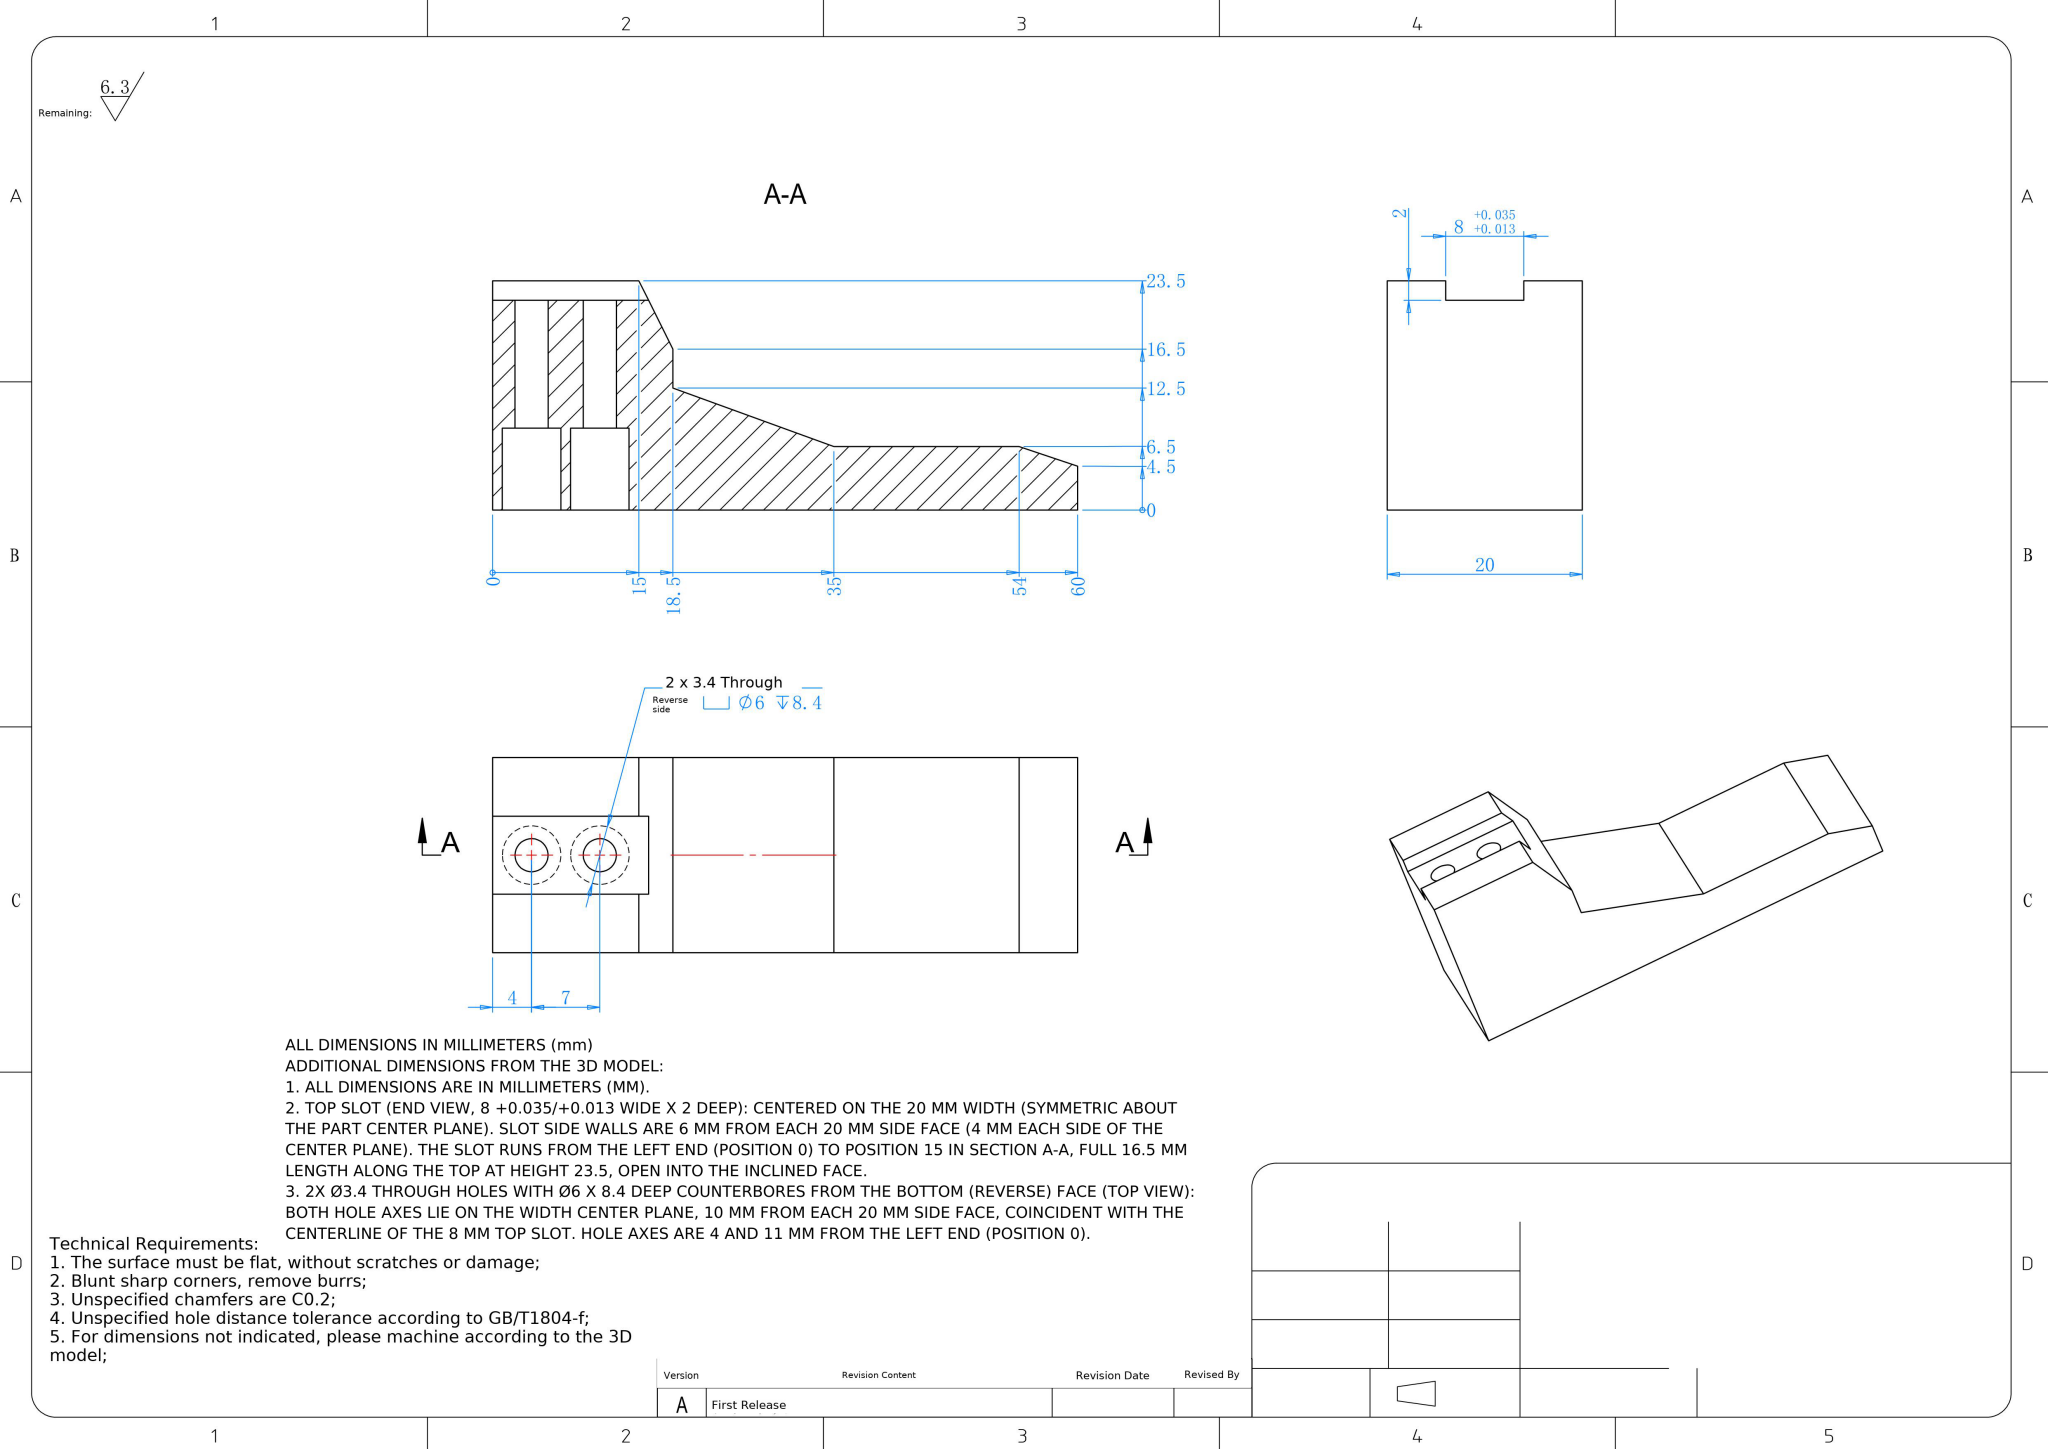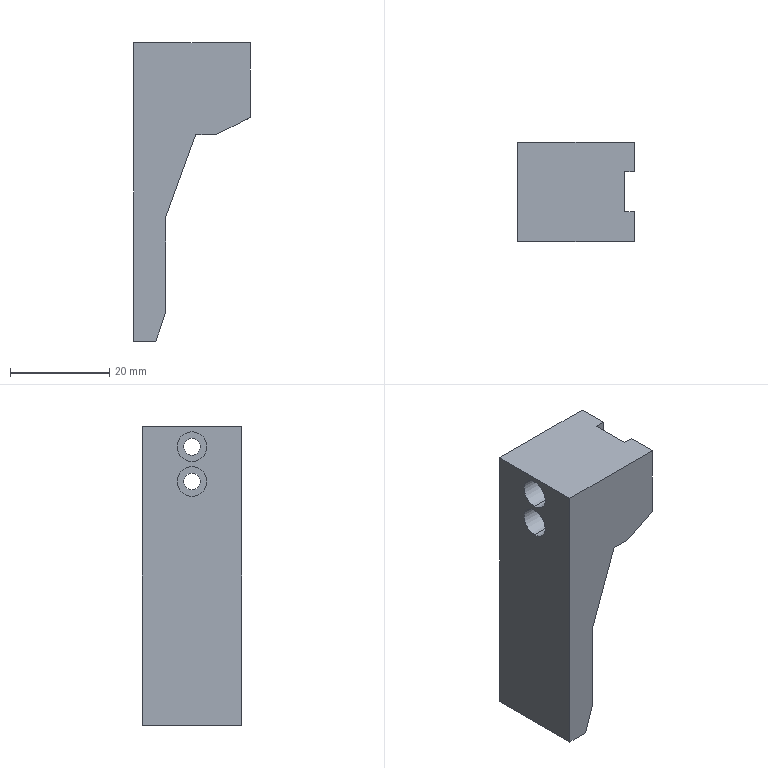Part | NX | mm | Stepped Dual-Bore Angled Mounting Bracket | 1 solid | 25 faces | box 23.5 x 20 x 60 mm | volume 13754 mm3 | plane 17 | cylinder 8 | commonest cylinder face diameters 6 x4 3.4 x4
STEP:
#1=COLOUR_RGB('',0.7922,0.8196,0.9333);
#2=FILL_AREA_STYLE_COLOUR('',#1);
#3=FILL_AREA_STYLE('',(#2));
#4=SURFACE_STYLE_FILL_AREA(#3);
#5=SURFACE_SIDE_STYLE('',(#4));
#6=SURFACE_STYLE_USAGE(.BOTH.,#5);
#7=PRESENTATION_STYLE_ASSIGNMENT((#6));
#8=CARTESIAN_POINT('',(8.4,0.,41.));
#9=VERTEX_POINT('',#8);
#10=CARTESIAN_POINT('',(8.4,0.,47.));
#11=VERTEX_POINT('',#10);
#12=CARTESIAN_POINT('',(8.4,0.,44.));
#13=DIRECTION('',(-1.,0.,0.));
#14=DIRECTION('',(0.,0.,1.));
#15=AXIS2_PLACEMENT_3D('',#12,#13,#14);
#16=CIRCLE('',#15,3.);
#17=EDGE_CURVE('',#9,#11,#16,.T.);
#18=ORIENTED_EDGE('',*,*,#17,.F.);
#19=CARTESIAN_POINT('',(0.,0.,41.));
#20=VERTEX_POINT('',#19);
#21=CARTESIAN_POINT('',(0.,0.,41.));
#22=DIRECTION('',(-1.,0.,0.));
#23=VECTOR('',#22,1000.);
#24=LINE('',#21,#23);
#25=EDGE_CURVE('',#9,#20,#24,.T.);
#26=ORIENTED_EDGE('',*,*,#25,.T.);
#27=CARTESIAN_POINT('',(0.,0.,47.));
#28=VERTEX_POINT('',#27);
#29=CARTESIAN_POINT('',(0.,0.,44.));
#30=DIRECTION('',(-1.,0.,0.));
#31=DIRECTION('',(0.,0.,1.));
#32=AXIS2_PLACEMENT_3D('',#29,#30,#31);
#33=CIRCLE('',#32,3.);
#34=EDGE_CURVE('',#20,#28,#33,.T.);
#35=ORIENTED_EDGE('',*,*,#34,.T.);
#36=CARTESIAN_POINT('',(0.,0.,47.));
#37=DIRECTION('',(-1.,0.,0.));
#38=VECTOR('',#37,1000.);
#39=LINE('',#36,#38);
#40=EDGE_CURVE('',#11,#28,#39,.T.);
#41=ORIENTED_EDGE('',*,*,#40,.F.);
#42=EDGE_LOOP('',(#18,#26,#35,#41));
#43=FACE_OUTER_BOUND('',#42,.T.);
#44=CARTESIAN_POINT('',(0.,0.,44.));
#45=DIRECTION('',(-1.,0.,0.));
#46=DIRECTION('',(0.,0.,1.));
#47=AXIS2_PLACEMENT_3D('',#44,#45,#46);
#48=CYLINDRICAL_SURFACE('',#47,3.);
#49=ADVANCED_FACE('',(#43),#48,.F.);
#50=CARTESIAN_POINT('',(21.5,0.,42.3));
#51=VERTEX_POINT('',#50);
#52=CARTESIAN_POINT('',(21.5,0.,45.7));
#53=VERTEX_POINT('',#52);
#54=CARTESIAN_POINT('',(21.5,0.,44.));
#55=DIRECTION('',(-1.,0.,0.));
#56=DIRECTION('',(0.,0.,1.));
#57=AXIS2_PLACEMENT_3D('',#54,#55,#56);
#58=CIRCLE('',#57,1.7);
#59=EDGE_CURVE('',#51,#53,#58,.T.);
#60=ORIENTED_EDGE('',*,*,#59,.F.);
#61=CARTESIAN_POINT('',(8.4,0.,42.3));
#62=VERTEX_POINT('',#61);
#63=CARTESIAN_POINT('',(0.,0.,42.3));
#64=DIRECTION('',(-1.,0.,0.));
#65=VECTOR('',#64,1000.);
#66=LINE('',#63,#65);
#67=EDGE_CURVE('',#51,#62,#66,.T.);
#68=ORIENTED_EDGE('',*,*,#67,.T.);
#69=CARTESIAN_POINT('',(8.4,0.,45.7));
#70=VERTEX_POINT('',#69);
#71=CARTESIAN_POINT('',(8.4,0.,44.));
#72=DIRECTION('',(-1.,0.,0.));
#73=DIRECTION('',(0.,0.,1.));
#74=AXIS2_PLACEMENT_3D('',#71,#72,#73);
#75=CIRCLE('',#74,1.7);
#76=EDGE_CURVE('',#62,#70,#75,.T.);
#77=ORIENTED_EDGE('',*,*,#76,.T.);
#78=CARTESIAN_POINT('',(0.,0.,45.7));
#79=DIRECTION('',(-1.,0.,0.));
#80=VECTOR('',#79,1000.);
#81=LINE('',#78,#80);
#82=EDGE_CURVE('',#53,#70,#81,.T.);
#83=ORIENTED_EDGE('',*,*,#82,.F.);
#84=EDGE_LOOP('',(#60,#68,#77,#83));
#85=FACE_OUTER_BOUND('',#84,.T.);
#86=CARTESIAN_POINT('',(0.,0.,44.));
#87=DIRECTION('',(-1.,0.,0.));
#88=DIRECTION('',(0.,0.,1.));
#89=AXIS2_PLACEMENT_3D('',#86,#87,#88);
#90=CYLINDRICAL_SURFACE('',#89,1.7);
#91=ADVANCED_FACE('',(#85),#90,.F.);
#92=CARTESIAN_POINT('',(8.4,0.,34.));
#93=VERTEX_POINT('',#92);
#94=CARTESIAN_POINT('',(8.4,0.,40.));
#95=VERTEX_POINT('',#94);
#96=CARTESIAN_POINT('',(8.4,0.,37.));
#97=DIRECTION('',(-1.,0.,0.));
#98=DIRECTION('',(0.,0.,1.));
#99=AXIS2_PLACEMENT_3D('',#96,#97,#98);
#100=CIRCLE('',#99,3.);
#101=EDGE_CURVE('',#93,#95,#100,.T.);
#102=ORIENTED_EDGE('',*,*,#101,.F.);
#103=CARTESIAN_POINT('',(0.,0.,34.));
#104=VERTEX_POINT('',#103);
#105=CARTESIAN_POINT('',(0.,0.,34.));
#106=DIRECTION('',(-1.,0.,0.));
#107=VECTOR('',#106,1000.);
#108=LINE('',#105,#107);
#109=EDGE_CURVE('',#93,#104,#108,.T.);
#110=ORIENTED_EDGE('',*,*,#109,.T.);
#111=CARTESIAN_POINT('',(0.,0.,40.));
#112=VERTEX_POINT('',#111);
#113=CARTESIAN_POINT('',(0.,0.,37.));
#114=DIRECTION('',(-1.,0.,0.));
#115=DIRECTION('',(0.,0.,1.));
#116=AXIS2_PLACEMENT_3D('',#113,#114,#115);
#117=CIRCLE('',#116,3.);
#118=EDGE_CURVE('',#104,#112,#117,.T.);
#119=ORIENTED_EDGE('',*,*,#118,.T.);
#120=CARTESIAN_POINT('',(0.,0.,40.));
#121=DIRECTION('',(-1.,0.,0.));
#122=VECTOR('',#121,1000.);
#123=LINE('',#120,#122);
#124=EDGE_CURVE('',#95,#112,#123,.T.);
#125=ORIENTED_EDGE('',*,*,#124,.F.);
#126=EDGE_LOOP('',(#102,#110,#119,#125));
#127=FACE_OUTER_BOUND('',#126,.T.);
#128=CARTESIAN_POINT('',(0.,0.,37.));
#129=DIRECTION('',(-1.,0.,0.));
#130=DIRECTION('',(0.,0.,1.));
#131=AXIS2_PLACEMENT_3D('',#128,#129,#130);
#132=CYLINDRICAL_SURFACE('',#131,3.);
#133=ADVANCED_FACE('',(#127),#132,.F.);
#134=CARTESIAN_POINT('',(21.5,0.,35.3));
#135=VERTEX_POINT('',#134);
#136=CARTESIAN_POINT('',(21.5,0.,38.7));
#137=VERTEX_POINT('',#136);
#138=CARTESIAN_POINT('',(21.5,0.,37.));
#139=DIRECTION('',(-1.,0.,0.));
#140=DIRECTION('',(0.,0.,1.));
#141=AXIS2_PLACEMENT_3D('',#138,#139,#140);
#142=CIRCLE('',#141,1.7);
#143=EDGE_CURVE('',#135,#137,#142,.T.);
#144=ORIENTED_EDGE('',*,*,#143,.F.);
#145=CARTESIAN_POINT('',(8.4,0.,35.3));
#146=VERTEX_POINT('',#145);
#147=CARTESIAN_POINT('',(0.,0.,35.3));
#148=DIRECTION('',(-1.,0.,0.));
#149=VECTOR('',#148,1000.);
#150=LINE('',#147,#149);
#151=EDGE_CURVE('',#135,#146,#150,.T.);
#152=ORIENTED_EDGE('',*,*,#151,.T.);
#153=CARTESIAN_POINT('',(8.4,0.,38.7));
#154=VERTEX_POINT('',#153);
#155=CARTESIAN_POINT('',(8.4,0.,37.));
#156=DIRECTION('',(-1.,0.,0.));
#157=DIRECTION('',(0.,0.,1.));
#158=AXIS2_PLACEMENT_3D('',#155,#156,#157);
#159=CIRCLE('',#158,1.7);
#160=EDGE_CURVE('',#146,#154,#159,.T.);
#161=ORIENTED_EDGE('',*,*,#160,.T.);
#162=CARTESIAN_POINT('',(0.,0.,38.7));
#163=DIRECTION('',(-1.,0.,0.));
#164=VECTOR('',#163,1000.);
#165=LINE('',#162,#164);
#166=EDGE_CURVE('',#137,#154,#165,.T.);
#167=ORIENTED_EDGE('',*,*,#166,.F.);
#168=EDGE_LOOP('',(#144,#152,#161,#167));
#169=FACE_OUTER_BOUND('',#168,.T.);
#170=CARTESIAN_POINT('',(0.,0.,37.));
#171=DIRECTION('',(-1.,0.,0.));
#172=DIRECTION('',(0.,0.,1.));
#173=AXIS2_PLACEMENT_3D('',#170,#171,#172);
#174=CYLINDRICAL_SURFACE('',#173,1.7);
#175=ADVANCED_FACE('',(#169),#174,.F.);
#176=CARTESIAN_POINT('',(23.5,-4.,33.));
#177=VERTEX_POINT('',#176);
#178=CARTESIAN_POINT('',(23.5,-10.,33.));
#179=VERTEX_POINT('',#178);
#180=CARTESIAN_POINT('',(23.5,10.,33.));
#181=DIRECTION('',(0.,-1.,0.));
#182=VECTOR('',#181,1000.);
#183=LINE('',#180,#182);
#184=EDGE_CURVE('',#177,#179,#183,.T.);
#185=ORIENTED_EDGE('',*,*,#184,.F.);
#186=CARTESIAN_POINT('',(23.5,-4.,48.));
#187=VERTEX_POINT('',#186);
#188=CARTESIAN_POINT('',(23.5,-4.,33.));
#189=DIRECTION('',(0.,0.,1.));
#190=VECTOR('',#189,1000.);
#191=LINE('',#188,#190);
#192=EDGE_CURVE('',#177,#187,#191,.T.);
#193=ORIENTED_EDGE('',*,*,#192,.T.);
#194=CARTESIAN_POINT('',(23.5,-10.,48.));
#195=VERTEX_POINT('',#194);
#196=CARTESIAN_POINT('',(23.5,10.,48.));
#197=DIRECTION('',(0.,-1.,0.));
#198=VECTOR('',#197,1000.);
#199=LINE('',#196,#198);
#200=EDGE_CURVE('',#187,#195,#199,.T.);
#201=ORIENTED_EDGE('',*,*,#200,.T.);
#202=CARTESIAN_POINT('',(23.5,-10.,33.));
#203=DIRECTION('',(-0.,0.,-1.));
#204=VECTOR('',#203,1000.);
#205=LINE('',#202,#204);
#206=EDGE_CURVE('',#195,#179,#205,.T.);
#207=ORIENTED_EDGE('',*,*,#206,.T.);
#208=EDGE_LOOP('',(#185,#193,#201,#207));
#209=FACE_OUTER_BOUND('',#208,.T.);
#210=CARTESIAN_POINT('',(23.5,10.,33.));
#211=DIRECTION('',(-1.,0.,0.));
#212=DIRECTION('',(0.,0.,1.));
#213=AXIS2_PLACEMENT_3D('',#210,#211,#212);
#214=PLANE('',#213);
#215=ADVANCED_FACE('',(#209),#214,.F.);
#216=CARTESIAN_POINT('',(0.,0.,44.));
#217=DIRECTION('',(-1.,0.,0.));
#218=DIRECTION('',(0.,0.,1.));
#219=AXIS2_PLACEMENT_3D('',#216,#217,#218);
#220=CIRCLE('',#219,3.);
#221=EDGE_CURVE('',#28,#20,#220,.T.);
#222=ORIENTED_EDGE('',*,*,#221,.F.);
#223=ORIENTED_EDGE('',*,*,#34,.F.);
#224=EDGE_LOOP('',(#222,#223));
#225=FACE_BOUND('',#224,.T.);
#226=CARTESIAN_POINT('',(0.,0.,37.));
#227=DIRECTION('',(-1.,0.,0.));
#228=DIRECTION('',(0.,0.,1.));
#229=AXIS2_PLACEMENT_3D('',#226,#227,#228);
#230=CIRCLE('',#229,3.);
#231=EDGE_CURVE('',#112,#104,#230,.T.);
#232=ORIENTED_EDGE('',*,*,#231,.F.);
#233=ORIENTED_EDGE('',*,*,#118,.F.);
#234=EDGE_LOOP('',(#232,#233));
#235=FACE_BOUND('',#234,.T.);
#236=CARTESIAN_POINT('',(0.,-10.,-12.));
#237=VERTEX_POINT('',#236);
#238=CARTESIAN_POINT('',(0.,-10.,48.));
#239=VERTEX_POINT('',#238);
#240=CARTESIAN_POINT('',(0.,-10.,48.));
#241=DIRECTION('',(0.,0.,1.));
#242=VECTOR('',#241,1000.);
#243=LINE('',#240,#242);
#244=EDGE_CURVE('',#237,#239,#243,.T.);
#245=ORIENTED_EDGE('',*,*,#244,.T.);
#246=CARTESIAN_POINT('',(0.,10.,48.));
#247=VERTEX_POINT('',#246);
#248=CARTESIAN_POINT('',(0.,10.,48.));
#249=DIRECTION('',(0.,-1.,0.));
#250=VECTOR('',#249,1000.);
#251=LINE('',#248,#250);
#252=EDGE_CURVE('',#247,#239,#251,.T.);
#253=ORIENTED_EDGE('',*,*,#252,.F.);
#254=CARTESIAN_POINT('',(0.,10.,-12.));
#255=VERTEX_POINT('',#254);
#256=CARTESIAN_POINT('',(0.,10.,48.));
#257=DIRECTION('',(0.,0.,1.));
#258=VECTOR('',#257,1000.);
#259=LINE('',#256,#258);
#260=EDGE_CURVE('',#255,#247,#259,.T.);
#261=ORIENTED_EDGE('',*,*,#260,.F.);
#262=CARTESIAN_POINT('',(0.,10.,-12.));
#263=DIRECTION('',(0.,-1.,0.));
#264=VECTOR('',#263,1000.);
#265=LINE('',#262,#264);
#266=EDGE_CURVE('',#255,#237,#265,.T.);
#267=ORIENTED_EDGE('',*,*,#266,.T.);
#268=EDGE_LOOP('',(#245,#253,#261,#267));
#269=FACE_OUTER_BOUND('',#268,.T.);
#270=CARTESIAN_POINT('',(0.,10.,48.));
#271=DIRECTION('',(1.,0.,0.));
#272=DIRECTION('',(0.,0.,-1.));
#273=AXIS2_PLACEMENT_3D('',#270,#271,#272);
#274=PLANE('',#273);
#275=ADVANCED_FACE('',(#225,#235,#269),#274,.F.);
#276=ORIENTED_EDGE('',*,*,#200,.F.);
#277=CARTESIAN_POINT('',(21.5,-4.,48.));
#278=VERTEX_POINT('',#277);
#279=CARTESIAN_POINT('',(21.5,-4.,48.));
#280=DIRECTION('',(1.,0.,0.));
#281=VECTOR('',#280,1000.);
#282=LINE('',#279,#281);
#283=EDGE_CURVE('',#278,#187,#282,.T.);
#284=ORIENTED_EDGE('',*,*,#283,.F.);
#285=CARTESIAN_POINT('',(21.5,4.,48.));
#286=VERTEX_POINT('',#285);
#287=CARTESIAN_POINT('',(21.5,-4.,48.));
#288=DIRECTION('',(0.,-1.,0.));
#289=VECTOR('',#288,1000.);
#290=LINE('',#287,#289);
#291=EDGE_CURVE('',#286,#278,#290,.T.);
#292=ORIENTED_EDGE('',*,*,#291,.F.);
#293=CARTESIAN_POINT('',(23.5,4.,48.));
#294=VERTEX_POINT('',#293);
#295=CARTESIAN_POINT('',(21.5,4.,48.));
#296=DIRECTION('',(-1.,0.,0.));
#297=VECTOR('',#296,1000.);
#298=LINE('',#295,#297);
#299=EDGE_CURVE('',#294,#286,#298,.T.);
#300=ORIENTED_EDGE('',*,*,#299,.F.);
#301=CARTESIAN_POINT('',(23.5,10.,48.));
#302=VERTEX_POINT('',#301);
#303=CARTESIAN_POINT('',(23.5,10.,48.));
#304=DIRECTION('',(0.,-1.,0.));
#305=VECTOR('',#304,1000.);
#306=LINE('',#303,#305);
#307=EDGE_CURVE('',#302,#294,#306,.T.);
#308=ORIENTED_EDGE('',*,*,#307,.F.);
#309=CARTESIAN_POINT('',(23.5,10.,48.));
#310=DIRECTION('',(1.,0.,0.));
#311=VECTOR('',#310,1000.);
#312=LINE('',#309,#311);
#313=EDGE_CURVE('',#247,#302,#312,.T.);
#314=ORIENTED_EDGE('',*,*,#313,.F.);
#315=ORIENTED_EDGE('',*,*,#252,.T.);
#316=CARTESIAN_POINT('',(23.5,-10.,48.));
#317=DIRECTION('',(1.,0.,0.));
#318=VECTOR('',#317,1000.);
#319=LINE('',#316,#318);
#320=EDGE_CURVE('',#239,#195,#319,.T.);
#321=ORIENTED_EDGE('',*,*,#320,.T.);
#322=EDGE_LOOP('',(#276,#284,#292,#300,#308,#314,#315,#321));
#323=FACE_OUTER_BOUND('',#322,.T.);
#324=CARTESIAN_POINT('',(23.5,10.,48.));
#325=DIRECTION('',(0.,0.,-1.));
#326=DIRECTION('',(-1.,0.,0.));
#327=AXIS2_PLACEMENT_3D('',#324,#325,#326);
#328=PLANE('',#327);
#329=ADVANCED_FACE('',(#323),#328,.F.);
#330=ORIENTED_EDGE('',*,*,#307,.T.);
#331=CARTESIAN_POINT('',(23.5,4.,33.));
#332=VERTEX_POINT('',#331);
#333=CARTESIAN_POINT('',(23.5,4.,33.));
#334=DIRECTION('',(-0.,0.,-1.));
#335=VECTOR('',#334,1000.);
#336=LINE('',#333,#335);
#337=EDGE_CURVE('',#294,#332,#336,.T.);
#338=ORIENTED_EDGE('',*,*,#337,.T.);
#339=CARTESIAN_POINT('',(23.5,10.,33.));
#340=VERTEX_POINT('',#339);
#341=CARTESIAN_POINT('',(23.5,10.,33.));
#342=DIRECTION('',(0.,-1.,0.));
#343=VECTOR('',#342,1000.);
#344=LINE('',#341,#343);
#345=EDGE_CURVE('',#340,#332,#344,.T.);
#346=ORIENTED_EDGE('',*,*,#345,.F.);
#347=CARTESIAN_POINT('',(23.5,10.,33.));
#348=DIRECTION('',(-0.,0.,-1.));
#349=VECTOR('',#348,1000.);
#350=LINE('',#347,#349);
#351=EDGE_CURVE('',#302,#340,#350,.T.);
#352=ORIENTED_EDGE('',*,*,#351,.F.);
#353=EDGE_LOOP('',(#330,#338,#346,#352));
#354=FACE_OUTER_BOUND('',#353,.T.);
#355=CARTESIAN_POINT('',(23.5,10.,33.));
#356=DIRECTION('',(-1.,0.,0.));
#357=DIRECTION('',(0.,0.,1.));
#358=AXIS2_PLACEMENT_3D('',#355,#356,#357);
#359=PLANE('',#358);
#360=ADVANCED_FACE('',(#354),#359,.F.);
#361=CARTESIAN_POINT('',(21.5,4.,32.));
#362=VERTEX_POINT('',#361);
#363=CARTESIAN_POINT('',(21.5,-4.,32.));
#364=VERTEX_POINT('',#363);
#365=CARTESIAN_POINT('',(21.5,10.,32.));
#366=DIRECTION('',(0.,-1.,0.));
#367=VECTOR('',#366,1000.);
#368=LINE('',#365,#367);
#369=EDGE_CURVE('',#362,#364,#368,.T.);
#370=ORIENTED_EDGE('',*,*,#369,.T.);
#371=CARTESIAN_POINT('',(23.5,-4.,33.));
#372=DIRECTION('',(0.8944,0.,0.4472));
#373=VECTOR('',#372,1000.);
#374=LINE('',#371,#373);
#375=EDGE_CURVE('',#364,#177,#374,.T.);
#376=ORIENTED_EDGE('',*,*,#375,.T.);
#377=ORIENTED_EDGE('',*,*,#184,.T.);
#378=CARTESIAN_POINT('',(16.5,-10.,29.5));
#379=VERTEX_POINT('',#378);
#380=CARTESIAN_POINT('',(23.5,-10.,33.));
#381=DIRECTION('',(-0.8944,0.,-0.4472));
#382=VECTOR('',#381,1000.);
#383=LINE('',#380,#382);
#384=EDGE_CURVE('',#179,#379,#383,.T.);
#385=ORIENTED_EDGE('',*,*,#384,.T.);
#386=CARTESIAN_POINT('',(16.5,10.,29.5));
#387=VERTEX_POINT('',#386);
#388=CARTESIAN_POINT('',(16.5,10.,29.5));
#389=DIRECTION('',(0.,-1.,0.));
#390=VECTOR('',#389,1000.);
#391=LINE('',#388,#390);
#392=EDGE_CURVE('',#387,#379,#391,.T.);
#393=ORIENTED_EDGE('',*,*,#392,.F.);
#394=CARTESIAN_POINT('',(23.5,10.,33.));
#395=DIRECTION('',(-0.8944,0.,-0.4472));
#396=VECTOR('',#395,1000.);
#397=LINE('',#394,#396);
#398=EDGE_CURVE('',#340,#387,#397,.T.);
#399=ORIENTED_EDGE('',*,*,#398,.F.);
#400=ORIENTED_EDGE('',*,*,#345,.T.);
#401=CARTESIAN_POINT('',(23.5,4.,33.));
#402=DIRECTION('',(-0.8944,0.,-0.4472));
#403=VECTOR('',#402,1000.);
#404=LINE('',#401,#403);
#405=EDGE_CURVE('',#332,#362,#404,.T.);
#406=ORIENTED_EDGE('',*,*,#405,.T.);
#407=EDGE_LOOP('',(#370,#376,#377,#385,#393,#399,#400,#406));
#408=FACE_OUTER_BOUND('',#407,.T.);
#409=CARTESIAN_POINT('',(23.5,10.,33.));
#410=DIRECTION('',(-0.4472,0.,0.8944));
#411=DIRECTION('',(0.8944,0.,0.4472));
#412=AXIS2_PLACEMENT_3D('',#409,#410,#411);
#413=PLANE('',#412);
#414=ADVANCED_FACE('',(#408),#413,.F.);
#415=CARTESIAN_POINT('',(12.5,-10.,29.5));
#416=VERTEX_POINT('',#415);
#417=CARTESIAN_POINT('',(16.5,-10.,29.5));
#418=DIRECTION('',(-1.,0.,0.));
#419=VECTOR('',#418,1000.);
#420=LINE('',#417,#419);
#421=EDGE_CURVE('',#379,#416,#420,.T.);
#422=ORIENTED_EDGE('',*,*,#421,.T.);
#423=CARTESIAN_POINT('',(12.5,10.,29.5));
#424=VERTEX_POINT('',#423);
#425=CARTESIAN_POINT('',(12.5,10.,29.5));
#426=DIRECTION('',(0.,-1.,0.));
#427=VECTOR('',#426,1000.);
#428=LINE('',#425,#427);
#429=EDGE_CURVE('',#424,#416,#428,.T.);
#430=ORIENTED_EDGE('',*,*,#429,.F.);
#431=CARTESIAN_POINT('',(16.5,10.,29.5));
#432=DIRECTION('',(-1.,0.,0.));
#433=VECTOR('',#432,1000.);
#434=LINE('',#431,#433);
#435=EDGE_CURVE('',#387,#424,#434,.T.);
#436=ORIENTED_EDGE('',*,*,#435,.F.);
#437=ORIENTED_EDGE('',*,*,#392,.T.);
#438=EDGE_LOOP('',(#422,#430,#436,#437));
#439=FACE_OUTER_BOUND('',#438,.T.);
#440=CARTESIAN_POINT('',(16.5,10.,29.5));
#441=DIRECTION('',(0.,0.,1.));
#442=DIRECTION('',(1.,0.,0.));
#443=AXIS2_PLACEMENT_3D('',#440,#441,#442);
#444=PLANE('',#443);
#445=ADVANCED_FACE('',(#439),#444,.F.);
#446=CARTESIAN_POINT('',(6.5,-10.,13.));
#447=VERTEX_POINT('',#446);
#448=CARTESIAN_POINT('',(12.5,-10.,29.5));
#449=DIRECTION('',(-0.3417,0.,-0.9398));
#450=VECTOR('',#449,1000.);
#451=LINE('',#448,#450);
#452=EDGE_CURVE('',#416,#447,#451,.T.);
#453=ORIENTED_EDGE('',*,*,#452,.T.);
#454=CARTESIAN_POINT('',(6.5,10.,13.));
#455=VERTEX_POINT('',#454);
#456=CARTESIAN_POINT('',(6.5,10.,13.));
#457=DIRECTION('',(0.,-1.,0.));
#458=VECTOR('',#457,1000.);
#459=LINE('',#456,#458);
#460=EDGE_CURVE('',#455,#447,#459,.T.);
#461=ORIENTED_EDGE('',*,*,#460,.F.);
#462=CARTESIAN_POINT('',(12.5,10.,29.5));
#463=DIRECTION('',(-0.3417,0.,-0.9398));
#464=VECTOR('',#463,1000.);
#465=LINE('',#462,#464);
#466=EDGE_CURVE('',#424,#455,#465,.T.);
#467=ORIENTED_EDGE('',*,*,#466,.F.);
#468=ORIENTED_EDGE('',*,*,#429,.T.);
#469=EDGE_LOOP('',(#453,#461,#467,#468));
#470=FACE_OUTER_BOUND('',#469,.T.);
#471=CARTESIAN_POINT('',(12.5,10.,29.5));
#472=DIRECTION('',(-0.9398,0.,0.3417));
#473=DIRECTION('',(0.3417,0.,0.9398));
#474=AXIS2_PLACEMENT_3D('',#471,#472,#473);
#475=PLANE('',#474);
#476=ADVANCED_FACE('',(#470),#475,.F.);
#477=CARTESIAN_POINT('',(6.5,-10.,-6.));
#478=VERTEX_POINT('',#477);
#479=CARTESIAN_POINT('',(6.5,-10.,-12.));
#480=DIRECTION('',(0.,0.,-1.));
#481=VECTOR('',#480,1000.);
#482=LINE('',#479,#481);
#483=EDGE_CURVE('',#447,#478,#482,.T.);
#484=ORIENTED_EDGE('',*,*,#483,.T.);
#485=CARTESIAN_POINT('',(6.5,10.,-6.));
#486=VERTEX_POINT('',#485);
#487=CARTESIAN_POINT('',(6.5,10.,-6.));
#488=DIRECTION('',(0.,-1.,0.));
#489=VECTOR('',#488,1000.);
#490=LINE('',#487,#489);
#491=EDGE_CURVE('',#486,#478,#490,.T.);
#492=ORIENTED_EDGE('',*,*,#491,.F.);
#493=CARTESIAN_POINT('',(6.5,10.,-12.));
#494=DIRECTION('',(0.,0.,-1.));
#495=VECTOR('',#494,1000.);
#496=LINE('',#493,#495);
#497=EDGE_CURVE('',#455,#486,#496,.T.);
#498=ORIENTED_EDGE('',*,*,#497,.F.);
#499=ORIENTED_EDGE('',*,*,#460,.T.);
#500=EDGE_LOOP('',(#484,#492,#498,#499));
#501=FACE_OUTER_BOUND('',#500,.T.);
#502=CARTESIAN_POINT('',(6.5,10.,-12.));
#503=DIRECTION('',(-1.,0.,-0.));
#504=DIRECTION('',(-0.,0.,1.));
#505=AXIS2_PLACEMENT_3D('',#502,#503,#504);
#506=PLANE('',#505);
#507=ADVANCED_FACE('',(#501),#506,.F.);
#508=CARTESIAN_POINT('',(4.5,10.,-12.));
#509=VERTEX_POINT('',#508);
#510=CARTESIAN_POINT('',(0.,10.,-12.));
#511=DIRECTION('',(-1.,0.,0.));
#512=VECTOR('',#511,1000.);
#513=LINE('',#510,#512);
#514=EDGE_CURVE('',#509,#255,#513,.T.);
#515=ORIENTED_EDGE('',*,*,#514,.F.);
#516=CARTESIAN_POINT('',(4.5,-10.,-12.));
#517=VERTEX_POINT('',#516);
#518=CARTESIAN_POINT('',(4.5,10.,-12.));
#519=DIRECTION('',(0.,-1.,0.));
#520=VECTOR('',#519,1000.);
#521=LINE('',#518,#520);
#522=EDGE_CURVE('',#509,#517,#521,.T.);
#523=ORIENTED_EDGE('',*,*,#522,.T.);
#524=CARTESIAN_POINT('',(0.,-10.,-12.));
#525=DIRECTION('',(-1.,0.,0.));
#526=VECTOR('',#525,1000.);
#527=LINE('',#524,#526);
#528=EDGE_CURVE('',#517,#237,#527,.T.);
#529=ORIENTED_EDGE('',*,*,#528,.T.);
#530=ORIENTED_EDGE('',*,*,#266,.F.);
#531=EDGE_LOOP('',(#515,#523,#529,#530));
#532=FACE_OUTER_BOUND('',#531,.T.);
#533=CARTESIAN_POINT('',(0.,10.,-12.));
#534=DIRECTION('',(0.,0.,1.));
#535=DIRECTION('',(1.,0.,-0.));
#536=AXIS2_PLACEMENT_3D('',#533,#534,#535);
#537=PLANE('',#536);
#538=ADVANCED_FACE('',(#532),#537,.F.);
#539=ORIENTED_EDGE('',*,*,#497,.T.);
#540=CARTESIAN_POINT('',(4.5,10.,-12.));
#541=DIRECTION('',(-0.3162,0.,-0.9487));
#542=VECTOR('',#541,1000.);
#543=LINE('',#540,#542);
#544=EDGE_CURVE('',#486,#509,#543,.T.);
#545=ORIENTED_EDGE('',*,*,#544,.T.);
#546=ORIENTED_EDGE('',*,*,#514,.T.);
#547=ORIENTED_EDGE('',*,*,#260,.T.);
#548=ORIENTED_EDGE('',*,*,#313,.T.);
#549=ORIENTED_EDGE('',*,*,#351,.T.);
#550=ORIENTED_EDGE('',*,*,#398,.T.);
#551=ORIENTED_EDGE('',*,*,#435,.T.);
#552=ORIENTED_EDGE('',*,*,#466,.T.);
#553=EDGE_LOOP('',(#539,#545,#546,#547,#548,#549,#550,#551,#552));
#554=FACE_OUTER_BOUND('',#553,.T.);
#555=CARTESIAN_POINT('',(0.,10.,0.));
#556=DIRECTION('',(0.,-1.,0.));
#557=DIRECTION('',(0.,0.,-1.));
#558=AXIS2_PLACEMENT_3D('',#555,#556,#557);
#559=PLANE('',#558);
#560=ADVANCED_FACE('',(#554),#559,.F.);
#561=CARTESIAN_POINT('',(4.5,-10.,-12.));
#562=DIRECTION('',(-0.3162,0.,-0.9487));
#563=VECTOR('',#562,1000.);
#564=LINE('',#561,#563);
#565=EDGE_CURVE('',#478,#517,#564,.T.);
#566=ORIENTED_EDGE('',*,*,#565,.F.);
#567=ORIENTED_EDGE('',*,*,#483,.F.);
#568=ORIENTED_EDGE('',*,*,#452,.F.);
#569=ORIENTED_EDGE('',*,*,#421,.F.);
#570=ORIENTED_EDGE('',*,*,#384,.F.);
#571=ORIENTED_EDGE('',*,*,#206,.F.);
#572=ORIENTED_EDGE('',*,*,#320,.F.);
#573=ORIENTED_EDGE('',*,*,#244,.F.);
#574=ORIENTED_EDGE('',*,*,#528,.F.);
#575=EDGE_LOOP('',(#566,#567,#568,#569,#570,#571,#572,#573,#574));
#576=FACE_OUTER_BOUND('',#575,.T.);
#577=CARTESIAN_POINT('',(0.,-10.,0.));
#578=DIRECTION('',(0.,-1.,0.));
#579=DIRECTION('',(0.,0.,-1.));
#580=AXIS2_PLACEMENT_3D('',#577,#578,#579);
#581=PLANE('',#580);
#582=ADVANCED_FACE('',(#576),#581,.T.);
#583=ORIENTED_EDGE('',*,*,#375,.F.);
#584=CARTESIAN_POINT('',(21.5,-4.,-12.));
#585=DIRECTION('',(0.,0.,1.));
#586=VECTOR('',#585,1000.);
#587=LINE('',#584,#586);
#588=EDGE_CURVE('',#364,#278,#587,.T.);
#589=ORIENTED_EDGE('',*,*,#588,.T.);
#590=ORIENTED_EDGE('',*,*,#283,.T.);
#591=ORIENTED_EDGE('',*,*,#192,.F.);
#592=EDGE_LOOP('',(#583,#589,#590,#591));
#593=FACE_OUTER_BOUND('',#592,.T.);
#594=CARTESIAN_POINT('',(21.5,-4.,-12.));
#595=DIRECTION('',(0.,-1.,0.));
#596=DIRECTION('',(0.,0.,-1.));
#597=AXIS2_PLACEMENT_3D('',#594,#595,#596);
#598=PLANE('',#597);
#599=ADVANCED_FACE('',(#593),#598,.F.);
#600=CARTESIAN_POINT('',(21.5,0.,44.));
#601=DIRECTION('',(-1.,0.,0.));
#602=DIRECTION('',(0.,0.,1.));
#603=AXIS2_PLACEMENT_3D('',#600,#601,#602);
#604=CIRCLE('',#603,1.7);
#605=EDGE_CURVE('',#53,#51,#604,.T.);
#606=ORIENTED_EDGE('',*,*,#605,.T.);
#607=ORIENTED_EDGE('',*,*,#59,.T.);
#608=EDGE_LOOP('',(#606,#607));
#609=FACE_BOUND('',#608,.T.);
#610=CARTESIAN_POINT('',(21.5,0.,37.));
#611=DIRECTION('',(-1.,0.,0.));
#612=DIRECTION('',(0.,0.,1.));
#613=AXIS2_PLACEMENT_3D('',#610,#611,#612);
#614=CIRCLE('',#613,1.7);
#615=EDGE_CURVE('',#137,#135,#614,.T.);
#616=ORIENTED_EDGE('',*,*,#615,.T.);
#617=ORIENTED_EDGE('',*,*,#143,.T.);
#618=EDGE_LOOP('',(#616,#617));
#619=FACE_BOUND('',#618,.T.);
#620=CARTESIAN_POINT('',(21.5,4.,-12.));
#621=DIRECTION('',(0.,0.,1.));
#622=VECTOR('',#621,1000.);
#623=LINE('',#620,#622);
#624=EDGE_CURVE('',#362,#286,#623,.T.);
#625=ORIENTED_EDGE('',*,*,#624,.T.);
#626=ORIENTED_EDGE('',*,*,#291,.T.);
#627=ORIENTED_EDGE('',*,*,#588,.F.);
#628=ORIENTED_EDGE('',*,*,#369,.F.);
#629=EDGE_LOOP('',(#625,#626,#627,#628));
#630=FACE_OUTER_BOUND('',#629,.T.);
#631=CARTESIAN_POINT('',(21.5,-4.,-12.));
#632=DIRECTION('',(-1.,0.,0.));
#633=DIRECTION('',(0.,0.,1.));
#634=AXIS2_PLACEMENT_3D('',#631,#632,#633);
#635=PLANE('',#634);
#636=ADVANCED_FACE('',(#609,#619,#630),#635,.F.);
#637=ORIENTED_EDGE('',*,*,#299,.T.);
#638=ORIENTED_EDGE('',*,*,#624,.F.);
#639=ORIENTED_EDGE('',*,*,#405,.F.);
#640=ORIENTED_EDGE('',*,*,#337,.F.);
#641=EDGE_LOOP('',(#637,#638,#639,#640));
#642=FACE_OUTER_BOUND('',#641,.T.);
#643=CARTESIAN_POINT('',(21.5,4.,-12.));
#644=DIRECTION('',(0.,1.,0.));
#645=DIRECTION('',(0.,0.,1.));
#646=AXIS2_PLACEMENT_3D('',#643,#644,#645);
#647=PLANE('',#646);
#648=ADVANCED_FACE('',(#642),#647,.F.);
#649=ORIENTED_EDGE('',*,*,#151,.F.);
#650=ORIENTED_EDGE('',*,*,#615,.F.);
#651=ORIENTED_EDGE('',*,*,#166,.T.);
#652=CARTESIAN_POINT('',(8.4,0.,37.));
#653=DIRECTION('',(-1.,0.,0.));
#654=DIRECTION('',(0.,0.,1.));
#655=AXIS2_PLACEMENT_3D('',#652,#653,#654);
#656=CIRCLE('',#655,1.7);
#657=EDGE_CURVE('',#154,#146,#656,.T.);
#658=ORIENTED_EDGE('',*,*,#657,.T.);
#659=EDGE_LOOP('',(#649,#650,#651,#658));
#660=FACE_OUTER_BOUND('',#659,.T.);
#661=CARTESIAN_POINT('',(0.,0.,37.));
#662=DIRECTION('',(-1.,0.,0.));
#663=DIRECTION('',(0.,0.,1.));
#664=AXIS2_PLACEMENT_3D('',#661,#662,#663);
#665=CYLINDRICAL_SURFACE('',#664,1.7);
#666=ADVANCED_FACE('',(#660),#665,.F.);
#667=ORIENTED_EDGE('',*,*,#657,.F.);
#668=ORIENTED_EDGE('',*,*,#160,.F.);
#669=EDGE_LOOP('',(#667,#668));
#670=FACE_BOUND('',#669,.T.);
#671=CARTESIAN_POINT('',(8.4,0.,37.));
#672=DIRECTION('',(-1.,0.,0.));
#673=DIRECTION('',(0.,0.,1.));
#674=AXIS2_PLACEMENT_3D('',#671,#672,#673);
#675=CIRCLE('',#674,3.);
#676=EDGE_CURVE('',#95,#93,#675,.T.);
#677=ORIENTED_EDGE('',*,*,#676,.T.);
#678=ORIENTED_EDGE('',*,*,#101,.T.);
#679=EDGE_LOOP('',(#677,#678));
#680=FACE_OUTER_BOUND('',#679,.T.);
#681=CARTESIAN_POINT('',(8.4,1.7,37.));
#682=DIRECTION('',(1.,0.,0.));
#683=DIRECTION('',(0.,0.,-1.));
#684=AXIS2_PLACEMENT_3D('',#681,#682,#683);
#685=PLANE('',#684);
#686=ADVANCED_FACE('',(#670,#680),#685,.F.);
#687=ORIENTED_EDGE('',*,*,#109,.F.);
#688=ORIENTED_EDGE('',*,*,#676,.F.);
#689=ORIENTED_EDGE('',*,*,#124,.T.);
#690=ORIENTED_EDGE('',*,*,#231,.T.);
#691=EDGE_LOOP('',(#687,#688,#689,#690));
#692=FACE_OUTER_BOUND('',#691,.T.);
#693=CARTESIAN_POINT('',(0.,0.,37.));
#694=DIRECTION('',(-1.,0.,0.));
#695=DIRECTION('',(0.,0.,1.));
#696=AXIS2_PLACEMENT_3D('',#693,#694,#695);
#697=CYLINDRICAL_SURFACE('',#696,3.);
#698=ADVANCED_FACE('',(#692),#697,.F.);
#699=ORIENTED_EDGE('',*,*,#67,.F.);
#700=ORIENTED_EDGE('',*,*,#605,.F.);
#701=ORIENTED_EDGE('',*,*,#82,.T.);
#702=CARTESIAN_POINT('',(8.4,0.,44.));
#703=DIRECTION('',(-1.,0.,0.));
#704=DIRECTION('',(0.,0.,1.));
#705=AXIS2_PLACEMENT_3D('',#702,#703,#704);
#706=CIRCLE('',#705,1.7);
#707=EDGE_CURVE('',#70,#62,#706,.T.);
#708=ORIENTED_EDGE('',*,*,#707,.T.);
#709=EDGE_LOOP('',(#699,#700,#701,#708));
#710=FACE_OUTER_BOUND('',#709,.T.);
#711=CARTESIAN_POINT('',(0.,0.,44.));
#712=DIRECTION('',(-1.,0.,0.));
#713=DIRECTION('',(0.,0.,1.));
#714=AXIS2_PLACEMENT_3D('',#711,#712,#713);
#715=CYLINDRICAL_SURFACE('',#714,1.7);
#716=ADVANCED_FACE('',(#710),#715,.F.);
#717=ORIENTED_EDGE('',*,*,#707,.F.);
#718=ORIENTED_EDGE('',*,*,#76,.F.);
#719=EDGE_LOOP('',(#717,#718));
#720=FACE_BOUND('',#719,.T.);
#721=CARTESIAN_POINT('',(8.4,0.,44.));
#722=DIRECTION('',(-1.,0.,0.));
#723=DIRECTION('',(0.,0.,1.));
#724=AXIS2_PLACEMENT_3D('',#721,#722,#723);
#725=CIRCLE('',#724,3.);
#726=EDGE_CURVE('',#11,#9,#725,.T.);
#727=ORIENTED_EDGE('',*,*,#726,.T.);
#728=ORIENTED_EDGE('',*,*,#17,.T.);
#729=EDGE_LOOP('',(#727,#728));
#730=FACE_OUTER_BOUND('',#729,.T.);
#731=CARTESIAN_POINT('',(8.4,1.7,44.));
#732=DIRECTION('',(1.,0.,0.));
#733=DIRECTION('',(0.,0.,-1.));
#734=AXIS2_PLACEMENT_3D('',#731,#732,#733);
#735=PLANE('',#734);
#736=ADVANCED_FACE('',(#720,#730),#735,.F.);
#737=ORIENTED_EDGE('',*,*,#25,.F.);
#738=ORIENTED_EDGE('',*,*,#726,.F.);
#739=ORIENTED_EDGE('',*,*,#40,.T.);
#740=ORIENTED_EDGE('',*,*,#221,.T.);
#741=EDGE_LOOP('',(#737,#738,#739,#740));
#742=FACE_OUTER_BOUND('',#741,.T.);
#743=CARTESIAN_POINT('',(0.,0.,44.));
#744=DIRECTION('',(-1.,0.,0.));
#745=DIRECTION('',(0.,0.,1.));
#746=AXIS2_PLACEMENT_3D('',#743,#744,#745);
#747=CYLINDRICAL_SURFACE('',#746,3.);
#748=ADVANCED_FACE('',(#742),#747,.F.);
#749=ORIENTED_EDGE('',*,*,#565,.T.);
#750=ORIENTED_EDGE('',*,*,#522,.F.);
#751=ORIENTED_EDGE('',*,*,#544,.F.);
#752=ORIENTED_EDGE('',*,*,#491,.T.);
#753=EDGE_LOOP('',(#749,#750,#751,#752));
#754=FACE_OUTER_BOUND('',#753,.T.);
#755=CARTESIAN_POINT('',(4.5,10.,-12.));
#756=DIRECTION('',(-0.9487,0.,0.3162));
#757=DIRECTION('',(0.3162,0.,0.9487));
#758=AXIS2_PLACEMENT_3D('',#755,#756,#757);
#759=PLANE('',#758);
#760=ADVANCED_FACE('',(#754),#759,.F.);
#761=CLOSED_SHELL('',(#49,#91,#133,#175,#215,#275,#329,#360,#414,#445,#476,#507,#538,#560,#582,#599,#636,#648,#666,#686,#698,#716,#736,#748,#760));
#762=MANIFOLD_SOLID_BREP('',#761);
#763=STYLED_ITEM('',(#7),#762);
#764=(LENGTH_UNIT()NAMED_UNIT(*)SI_UNIT(.MILLI.,.METRE.));
#765=UNCERTAINTY_MEASURE_WITH_UNIT(LENGTH_MEASURE(0.00001),#764,'','');
#766=(NAMED_UNIT(*)PLANE_ANGLE_UNIT()SI_UNIT($,.RADIAN.));
#767=(NAMED_UNIT(*)SI_UNIT($,.STERADIAN.)SOLID_ANGLE_UNIT());
#768=(GEOMETRIC_REPRESENTATION_CONTEXT(3)GLOBAL_UNCERTAINTY_ASSIGNED_CONTEXT((#765))GLOBAL_UNIT_ASSIGNED_CONTEXT((#764,#766,#767))REPRESENTATION_CONTEXT('',''));
#769=MECHANICAL_DESIGN_GEOMETRIC_PRESENTATION_REPRESENTATION('',(#763),#768);
#770=CARTESIAN_POINT('',(0.,0.,0.));
#771=DIRECTION('',(0.,0.,1.));
#772=DIRECTION('',(1.,0.,0.));
#773=AXIS2_PLACEMENT_3D('',#770,#771,#772);
#774=(LENGTH_UNIT()NAMED_UNIT(*)SI_UNIT(.MILLI.,.METRE.));
#775=UNCERTAINTY_MEASURE_WITH_UNIT(LENGTH_MEASURE(0.00001),#774,'','');
#776=(NAMED_UNIT(*)PLANE_ANGLE_UNIT()SI_UNIT($,.RADIAN.));
#777=(NAMED_UNIT(*)SI_UNIT($,.STERADIAN.)SOLID_ANGLE_UNIT());
#778=(GEOMETRIC_REPRESENTATION_CONTEXT(3)GLOBAL_UNCERTAINTY_ASSIGNED_CONTEXT((#775))GLOBAL_UNIT_ASSIGNED_CONTEXT((#774,#776,#777))REPRESENTATION_CONTEXT('',''));
#779=ADVANCED_BREP_SHAPE_REPRESENTATION('',(#762,#773),#778);
#780=PRESENTATION_LAYER_ASSIGNMENT('','',(#763));